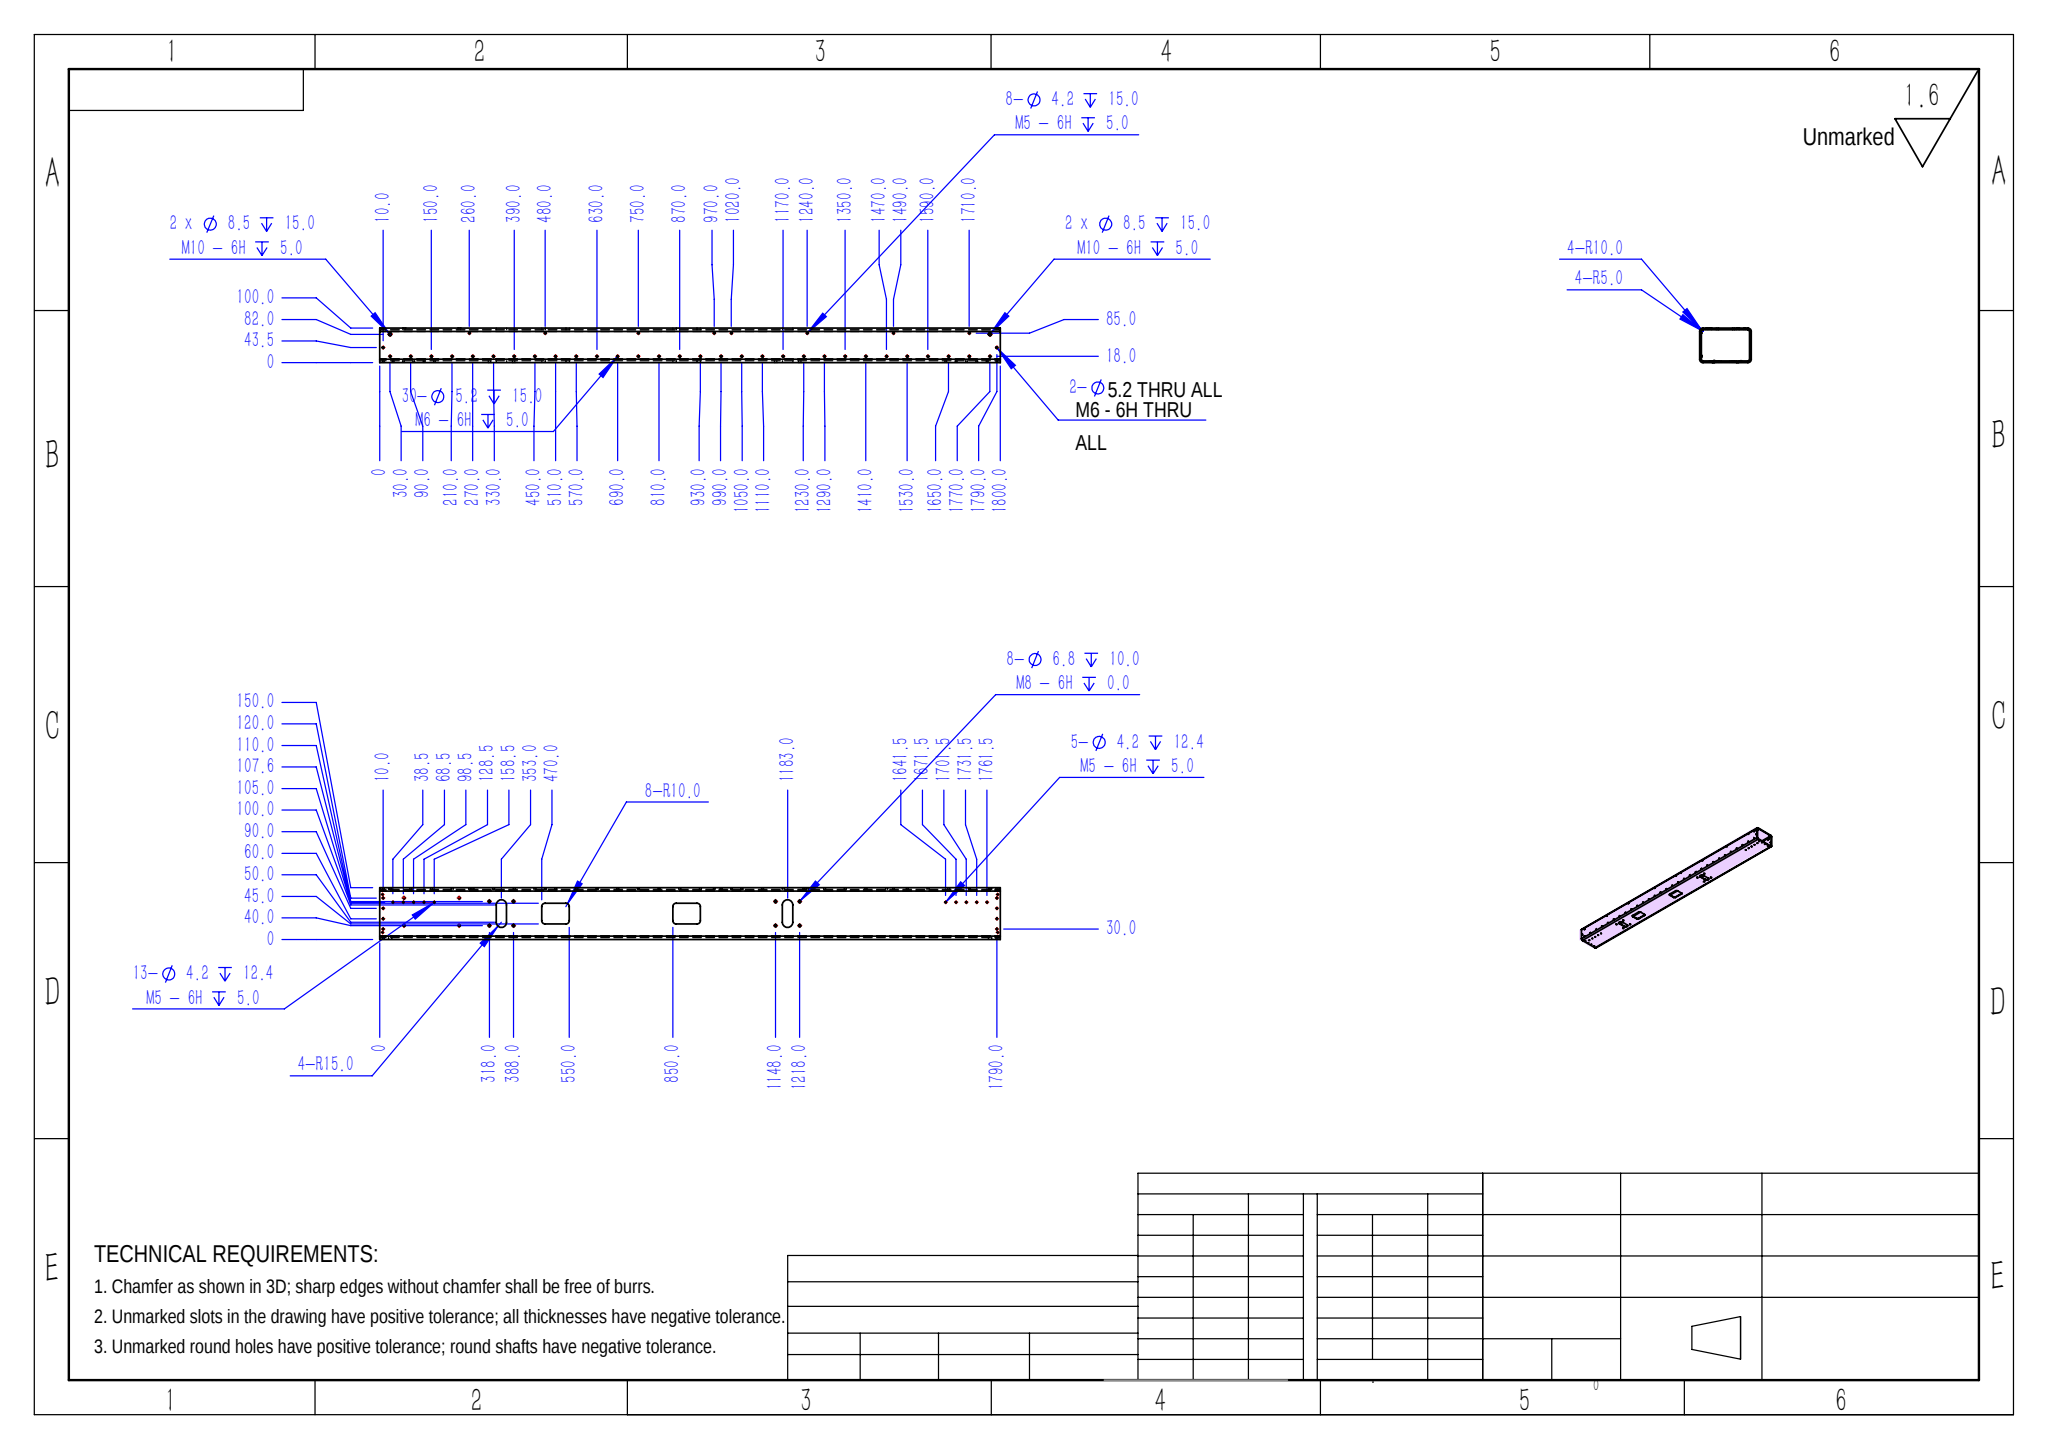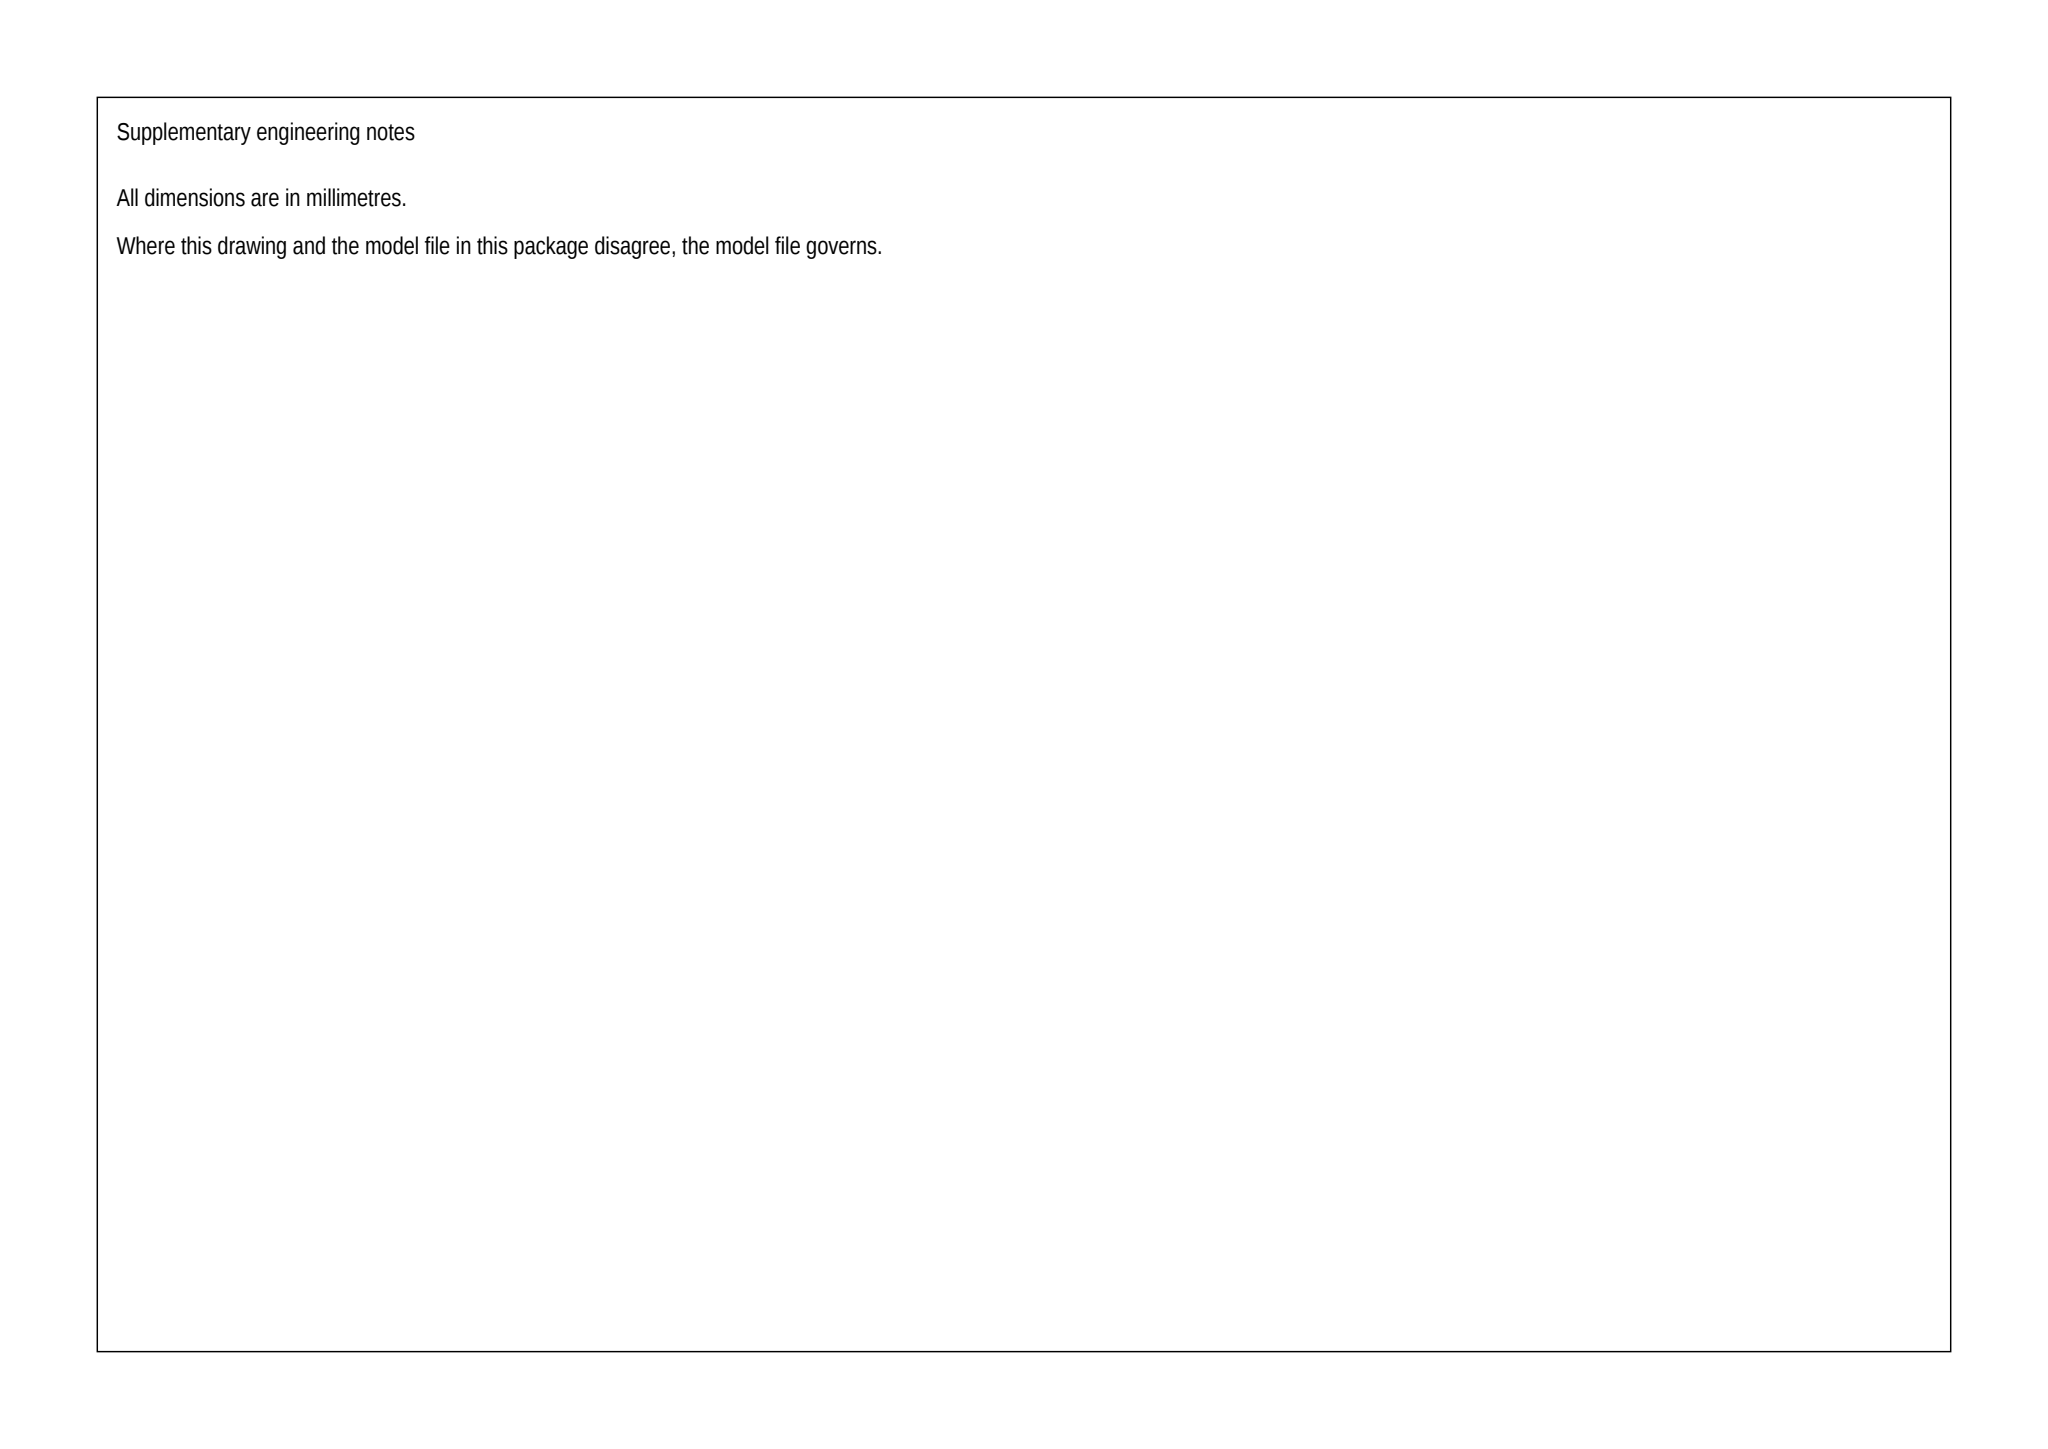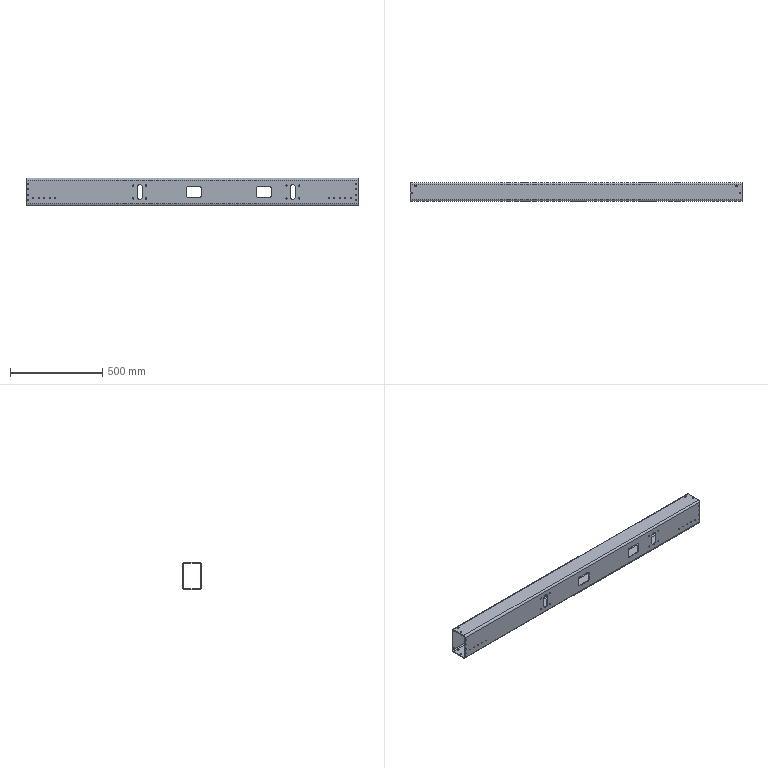Part | SolidWorks | mm | 1 solid | 226 faces | box 1800 x 100 x 150 mm | volume 4056692 mm3 | cylinder 192 | plane 34 | commonest cylinder face diameters 5.2 x68 4.2 x60 6.8 x24 20 x20 8.5 x8 30 x8 10 x4
Drawing notes:
SECT: 150 X 100 RECT TUBE, 1800 LG, WALL THK 5 ALL 4 SIDES | from the solid: bbox 1800x100x150; axis planes y=0/5/95/100 and z=0/5/145/150
4X Ø10 THRU 1800 LG, 10 FROM EA ADJACENT OUTER FACE | from the solid: cyl Ø10 axis x, len 1800 at (y,z)=(10,10),(10,140),(90,10),(90,140)
2X POCKET 80 LG X 60 HI, X 870-950 & 1250-1330, Z 45-105, THRU BOTH WALLS | from the solid: x planes 870/950 & 1250/1330 (cnt 2 ea); z planes 45/105 (cnt 4 ea); walls 5 THK
2X SIDE CUTOUT 30 LG X 60 HI, X 602-632 & 1432-1462, Z 45-105, THRU BOTH WALLS | from the solid: x planes 602/632 & 1432/1462 (cnt 2 ea); z planes 45/105; y planes 0,5,95,100
SIDE M5 ROWS X 38.5-158.5 & 1641.5-1761.5 AT Z=42.37 FROM BOT FACE | from the solid: Ø4.2 axis y at z=42.37, x=38.5..158.5 and 1641.5..1761.5
SIDE M5 AT X=10 & 1790: Z=30,60,90,120 FROM BOT FACE | from the solid: Ø4.2 axis y at x=10 & 1790, z=30,60,90,120
SIDE M5 AT X=8 & 1792: Z=20 & 130 FROM BOT FACE | from the solid: Ø4.2 axis y at x=8 & 1792, z=20 and 130
SIDE M8 (Ø6.8) AT X=582,652,1412,1482: Z=40 & 110 FROM BOT FACE | from the solid: Ø6.8 axis y at x=582,652,1412,1482, z=40 and 110
SIDE M8 (Ø6.8) AT X=1570 & 1730: Z=30 & 110 FROM BOT FACE | from the solid: Ø6.8 axis y at x=1570 & 1730, z=30 and 110
ALL SIDE-WALL HOLES 2X, BOTH WALLS (Y 0-5 & 95-100), DP 5 EA | from the solid: all axis-y cylinders count 2, length 5; walls y 0-5, 95-100
TOP 8X M5 AT Y=85: X=90,310,560,780,830,1050,1320,1540 | from the solid: Ø4.2 axis z at y=85, x=90,310,560,780,830,1050,1320,1540
ALL TOP-FACE HOLE PATTERNS REPEAT IN BTM WALL, DP 5 EA | from the solid: axis-z cylinders count 2 per position, length 5; walls z 0-5, 145-150
Ø5.2 DP 15 / M6-6H DP 5 AT X=10 & 1790: Y=43.5 & 56.5, TOP & BOT FACES | from the solid: cylinders [5.2,"z",[10.0,43.5,null],5.0,count 4] and [5.2,"z",[1790.0,43.5,null],5.0,count 4]; bbox Y=100 so mirrored row at Y=100-43.5=56.5; 4 per end = 2 Y-rows x 2 faces (z=0/150)
POCKETS 80x60 AT X=870 & 1250; CUTOUTS 30x60 AT X=602 & 1432 | from the solid: axis_planes x=870/950 & 1250/1330 (80 wide), x=602/632 & 1432/1462 (30 wide), z=45/105 count 4 (60 high)
build123d program:
from build123d import *

# Parameters (mm, degrees)
GB_6728_1986_RECTANGULAR_HOLLOW_SECTION_DEPTH = 1800
SKETCH2_W                                     = 80
SKETCH2_H                                     = 60
CUT_EXTRUDE1_DEPTH                            = 909.639
LPATTERN1_COUNT                               = 2
LPATTERN1_PITCH                               = 380
FILLET1_R                                     = 10
M6_TAPPED_HOLE1_D                             = 5.2
M5_TAPPED_HOLE1_AT_2_COUNT                    = 2
M5_TAPPED_HOLE1_AT_2_PITCH                    = 30
M5_TAPPED_HOLE1_AT_3_COUNT                    = 2
M5_TAPPED_HOLE1_AT_3_PITCH                    = 90
M5_TAPPED_HOLE1_AT_4_COUNT                    = 2
M5_TAPPED_HOLE1_AT_4_PITCH                    = 60
LPATTERN2_COUNT                               = 5
LPATTERN2_PITCH                               = 30
M10_TAPPED_HOLE1_D                            = 8.5
M10_TAPPED_HOLE1_DEPTH                        = 15
M10_TAPPED_HOLE1_TIP                          = 2.554
M8_TAPPED_HOLE3_D                             = 6.8
M8_TAPPED_HOLE3_DEPTH                         = 10
M8_TAPPED_HOLE3_TIP                           = 2.043
CUT_EXTRUDE2_DEPTH                            = 909.639
M5_TAPPED_HOLE5_D                             = 4.2
M5_TAPPED_HOLE5_DEPTH                         = 15
M5_TAPPED_HOLE5_TIP                           = 1.262
M6_TAPPED_HOLE2_D                             = 5.2
M6_TAPPED_HOLE2_DEPTH                         = 15
M6_TAPPED_HOLE2_TIP                           = 1.562
M8_TAPPED_HOLE5_D                             = 6.8
M8_TAPPED_HOLE5_DEPTH                         = 15
M8_TAPPED_HOLE5_TIP                           = 2.043
M5_TAPPED_HOLE6_AT_2_COUNT                    = 2
M5_TAPPED_HOLE6_AT_2_PITCH                    = 110


with BuildPart() as part:
    # Sketch11 → GB_6728-1986 Rectangular Hollow Section (new body)
    with BuildSketch(Plane.YZ.offset(-900)):
        with BuildLine():
            Line((-40, -75), (40, -75))
            ThreePointArc((40, -75), (47.071, -72.071), (50, -65))
            Line((50, -65), (50, 65))
            ThreePointArc((50, 65), (47.071, 72.071), (40, 75))
            Line((40, 75), (-40, 75))
            ThreePointArc((-40, 75), (-47.071, 72.071), (-50, 65))
            Line((-50, 65), (-50, -65))
            ThreePointArc((-50, -65), (-47.071, -72.071), (-40, -75))
        make_face()
        with BuildLine():
            Line((-40, -70), (40, -70))
            ThreePointArc((40, -70), (43.536, -68.536), (45, -65))
            Line((45, -65), (45, 65))
            ThreePointArc((45, 65), (43.536, 68.536), (40, 70))
            Line((40, 70), (-40, 70))
            ThreePointArc((-40, 70), (-43.536, 68.536), (-45, 65))
            Line((-45, 65), (-45, -65))
            ThreePointArc((-45, -65), (-43.536, -68.536), (-40, -70))
        make_face(mode=Mode.SUBTRACT)
    extrude(amount=GB_6728_1986_RECTANGULAR_HOLLOW_SECTION_DEPTH)

    # Sketch2 → Cut-Extrude1 (cut, through all)
    with BuildSketch(Plane.XZ.offset(50)):
        with Locations((390, 0)):
            Rectangle(SKETCH2_W, SKETCH2_H)
    cut_extrude1 = extrude(amount=-CUT_EXTRUDE1_DEPTH, mode=Mode.SUBTRACT)

    # LPattern1: Cut-Extrude1 ×2
    with Locations(*[(-i * LPATTERN1_PITCH, 0, 0) for i in range(1, LPATTERN1_COUNT)]):
        add(cut_extrude1, mode=Mode.SUBTRACT)

    # Fillet1
    fillet1_edges = [part.edges().sort_by_distance(p)[0] for p in [
        (430, 47.5, 30),
        (430, 47.5, -30),
        (350, 47.5, -30),
        (350, 47.5, 30),
        (430, -47.5, 30),
        (430, -47.5, -30),
        (350, -47.5, -30),
        (350, -47.5, 30),
        (50, 47.5, 30),
        (50, 47.5, -30),
        (-30, 47.5, -30),
        (-30, 47.5, 30),
        (50, -47.5, 30),
        (50, -47.5, -30),
        (-30, -47.5, -30),
        (-30, -47.5, 30),
    ]]
    fillet(fillet1_edges, radius=FILLET1_R)

    # M6 Tapped Hole1 (through all)
    with Locations(Plane.XY.offset(75)):
        with Locations((890, -6.5), (-890, -6.5)):
            Hole(M6_TAPPED_HOLE1_D / 2)

    # Sketch5 → M5 Tapped Hole1 (revolve, cut)
    with BuildSketch(Plane(origin=(890, -50, -45), x_dir=(0, 0, -1), z_dir=(1, 0, 0))):
        Polygon((0, 0), (0, 13.662), (2.1, 12.4), (2.1, 0), align=None)
    m5_tapped_hole1 = revolve(axis=Axis((890, -56.35, -45), (0, 1, 0)), mode=Mode.SUBTRACT)

    # M5 Tapped Hole1 at 2: M5 Tapped Hole1 ×2
    with Locations(*[(0, 0, i * M5_TAPPED_HOLE1_AT_2_PITCH) for i in range(1, M5_TAPPED_HOLE1_AT_2_COUNT)]):
        add(m5_tapped_hole1, mode=Mode.SUBTRACT)

    # M5 Tapped Hole1 at 3: M5 Tapped Hole1 ×2
    with Locations(*[(0, 0, i * M5_TAPPED_HOLE1_AT_3_PITCH) for i in range(1, M5_TAPPED_HOLE1_AT_3_COUNT)]):
        add(m5_tapped_hole1, mode=Mode.SUBTRACT)

    # M5 Tapped Hole1 at 4: M5 Tapped Hole1 ×2
    with Locations(*[(0, 0, i * M5_TAPPED_HOLE1_AT_4_PITCH) for i in range(1, M5_TAPPED_HOLE1_AT_4_COUNT)]):
        add(m5_tapped_hole1, mode=Mode.SUBTRACT)

    # Sketch8 → M5 Tapped Hole2 (revolve, cut)
    with BuildSketch(Plane(origin=(861.5, -50, -32.627), x_dir=(0, 0, -1), z_dir=(1, 0, 0))):
        Polygon((0, 0), (0, 13.662), (2.1, 12.4), (2.1, 0), align=None)
    m5_tapped_hole2 = revolve(axis=Axis((861.5, -56.35, -32.627), (0, 1, 0)), mode=Mode.SUBTRACT)

    # LPattern2: M5 Tapped Hole2 ×5
    with Locations(*[(-i * LPATTERN2_PITCH, 0, 0) for i in range(1, LPATTERN2_COUNT)]):
        add(m5_tapped_hole2, mode=Mode.SUBTRACT)

    # M10 Tapped Hole1
    with Locations(Plane(origin=(0, 0, 70), x_dir=(-1, 0, 0), z_dir=(0, 0, -1))):
        with Locations((-870, 32), (870, 32)):
            Hole(M10_TAPPED_HOLE1_D / 2, depth=M10_TAPPED_HOLE1_DEPTH)
            with Locations((0, 0, -(M10_TAPPED_HOLE1_DEPTH + M10_TAPPED_HOLE1_TIP / 2))):  # 118° drill point
                Cone(0, M10_TAPPED_HOLE1_D / 2, M10_TAPPED_HOLE1_TIP, mode=Mode.SUBTRACT)

    # Sketch11_2 → M10 Tapped Hole2 (revolve, cut)
    with BuildSketch(Plane(origin=(870, 32, -70), x_dir=(0, -1, 0), z_dir=(1, 0, 0))):
        Polygon((0, 0), (0, 17.554), (4.25, 15), (4.25, 0), align=None)
    m10_tapped_hole2 = revolve(axis=Axis((870, 32, -63.65), (0, 0, -1)), mode=Mode.SUBTRACT)

    # M8 Tapped Hole3
    with Locations(Plane(origin=(0, -50, 0), x_dir=(-1, 0, 0), z_dir=(0, -1, 0))):
        with Locations((-512, -35), (-582, -35), (-582, 35), (-512, 35), (318, -35), (248, -35), (248, 35), (318, 35)):
            Hole(M8_TAPPED_HOLE3_D / 2, depth=M8_TAPPED_HOLE3_DEPTH)
            with Locations((0, 0, -(M8_TAPPED_HOLE3_DEPTH + M8_TAPPED_HOLE3_TIP / 2))):  # 118° drill point
                Cone(0, M8_TAPPED_HOLE3_D / 2, M8_TAPPED_HOLE3_TIP, mode=Mode.SUBTRACT)

    # Sketch21 → Cut-Extrude2 (cut, through all)
    with BuildSketch(Plane.XZ.offset(50)):
        with BuildLine():
            Line((-298, 25), (-298, -25))
            ThreePointArc((-298, -25), (-283, -40), (-268, -25))
            Line((-268, -25), (-268, 25))
            ThreePointArc((-268, 25), (-283, 40), (-298, 25))
        make_face()
        with BuildLine():
            Line((532, 25), (532, -25))
            ThreePointArc((532, -25), (547, -40), (562, -25))
            Line((562, -25), (562, 25))
            ThreePointArc((562, 25), (547, 40), (532, 25))
        make_face()
    extrude(amount=-CUT_EXTRUDE2_DEPTH, mode=Mode.SUBTRACT)

    # Mirror1: M5 Tapped Hole2, M10 Tapped Hole2 across plane
    add(m5_tapped_hole2.mirror(Plane(origin=(0, 0, 0), x_dir=(0, 0, 1), z_dir=(1, 0, 0))), mode=Mode.SUBTRACT)
    add(m10_tapped_hole2.mirror(Plane(origin=(0, 0, 0), x_dir=(0, 0, 1), z_dir=(1, 0, 0))), mode=Mode.SUBTRACT)

    # Mirror1 copy 1 sketch → Mirror1 copy 1 (revolve, cut)
    with BuildSketch(Plane(origin=(-831.5, -50, -32.627), x_dir=(0, 0, -1), z_dir=(-1, 0, 0))):
        Polygon((0, 0), (0, -13.662), (2.1, -12.4), (2.1, 0), align=None)
    revolve(axis=Axis((-831.5, -56.35, -32.627), (0, -1, 0)), mode=Mode.SUBTRACT)

    # Mirror1 copy 2 sketch → Mirror1 copy 2 (revolve, cut)
    with BuildSketch(Plane(origin=(-801.5, -50, -32.627), x_dir=(0, 0, -1), z_dir=(-1, 0, 0))):
        Polygon((0, 0), (0, -13.662), (2.1, -12.4), (2.1, 0), align=None)
    revolve(axis=Axis((-801.5, -56.35, -32.627), (0, -1, 0)), mode=Mode.SUBTRACT)

    # Mirror1 copy 3 sketch → Mirror1 copy 3 (revolve, cut)
    with BuildSketch(Plane(origin=(-771.5, -50, -32.627), x_dir=(0, 0, -1), z_dir=(-1, 0, 0))):
        Polygon((0, 0), (0, -13.662), (2.1, -12.4), (2.1, 0), align=None)
    revolve(axis=Axis((-771.5, -56.35, -32.627), (0, -1, 0)), mode=Mode.SUBTRACT)

    # Mirror1 copy 4 sketch → Mirror1 copy 4 (revolve, cut)
    with BuildSketch(Plane(origin=(-741.5, -50, -32.627), x_dir=(0, 0, -1), z_dir=(-1, 0, 0))):
        Polygon((0, 0), (0, -13.662), (2.1, -12.4), (2.1, 0), align=None)
    revolve(axis=Axis((-741.5, -56.35, -32.627), (0, -1, 0)), mode=Mode.SUBTRACT)

    # M5 Tapped Hole5
    with Locations(Plane(origin=(0, 0, -75), x_dir=(-1, 0, 0), z_dir=(0, 0, -1))):
        with Locations((70, 35), (-150, 35), (-640, 35), (-420, 35), (810, 35), (590, 35), (120, 35), (340, 35)):
            Hole(M5_TAPPED_HOLE5_D / 2, depth=M5_TAPPED_HOLE5_DEPTH)
            with Locations((0, 0, -(M5_TAPPED_HOLE5_DEPTH + M5_TAPPED_HOLE5_TIP / 2))):  # 118° drill point
                Cone(0, M5_TAPPED_HOLE5_D / 2, M5_TAPPED_HOLE5_TIP, mode=Mode.SUBTRACT)

    # M6 Tapped Hole2
    with Locations(Plane(origin=(0, 0, -75), x_dir=(-1, 0, 0), z_dir=(0, 0, -1))):
        with Locations((870, -32), (-870, -32), (-810, -32), (-750, -32), (-690, -32), (-630, -32), (-570, -32), (-510, -32), (-450, -32), (-390, -32), (-330, -32), (-270, -32), (-210, -32), (-150, -32), (-90, -32), (-30, -32), (30, -32), (90, -32), (150, -32), (210, -32), (270, -32), (330, -32), (390, -32), (450, -32), (510, -32), (570, -32), (630, -32), (690, -32), (750, -32), (810, -32)):
            Hole(M6_TAPPED_HOLE2_D / 2, depth=M6_TAPPED_HOLE2_DEPTH)
            with Locations((0, 0, -(M6_TAPPED_HOLE2_DEPTH + M6_TAPPED_HOLE2_TIP / 2))):  # 118° drill point
                Cone(0, M6_TAPPED_HOLE2_D / 2, M6_TAPPED_HOLE2_TIP, mode=Mode.SUBTRACT)

    # M8 Tapped Hole5
    with Locations(Plane(origin=(0, 50, 0), x_dir=(1, 0, 0), z_dir=(0, 1, 0))):
        with Locations((670, 45), (670, -35), (830, 45), (830, -35)):
            Hole(M8_TAPPED_HOLE5_D / 2, depth=M8_TAPPED_HOLE5_DEPTH)
            with Locations((0, 0, -(M8_TAPPED_HOLE5_DEPTH + M8_TAPPED_HOLE5_TIP / 2))):  # 118° drill point
                Cone(0, M8_TAPPED_HOLE5_D / 2, M8_TAPPED_HOLE5_TIP, mode=Mode.SUBTRACT)

    # Mirror2: M5 Tapped Hole1 across plane
    add(m5_tapped_hole1.mirror(Plane(origin=(0, 0, 0), x_dir=(0, 0, 1), z_dir=(1, 0, 0))), mode=Mode.SUBTRACT)

    # Mirror2 copy 1 sketch → Mirror2 copy 1 (revolve, cut)
    with BuildSketch(Plane(origin=(-890, -50, -15), x_dir=(0, 0, -1), z_dir=(-1, 0, 0))):
        Polygon((0, 0), (0, -13.662), (2.1, -12.4), (2.1, 0), align=None)
    revolve(axis=Axis((-890, -56.35, -15), (0, -1, 0)), mode=Mode.SUBTRACT)

    # Mirror2 copy 2 sketch → Mirror2 copy 2 (revolve, cut)
    with BuildSketch(Plane(origin=(-890, -50, 45), x_dir=(0, 0, -1), z_dir=(-1, 0, 0))):
        Polygon((0, 0), (0, -13.662), (2.1, -12.4), (2.1, 0), align=None)
    revolve(axis=Axis((-890, -56.35, 45), (0, -1, 0)), mode=Mode.SUBTRACT)

    # Mirror2 copy 3 sketch → Mirror2 copy 3 (revolve, cut)
    with BuildSketch(Plane(origin=(-890, -50, 15), x_dir=(0, 0, -1), z_dir=(-1, 0, 0))):
        Polygon((0, 0), (0, -13.662), (2.1, -12.4), (2.1, 0), align=None)
    revolve(axis=Axis((-890, -56.35, 15), (0, -1, 0)), mode=Mode.SUBTRACT)

    # Sketch42 → M5 Tapped Hole6 (revolve, cut)
    with BuildSketch(Plane(origin=(892, 50, 55), x_dir=(0, 0, 1), z_dir=(1, 0, 0))):
        Polygon((0, 0), (0, 11.262), (2.1, 10), (2.1, 0), align=None)
    m5_tapped_hole6 = revolve(axis=Axis((892, 56.35, 55), (0, -1, 0)), mode=Mode.SUBTRACT)

    # M5 Tapped Hole6 at 2: M5 Tapped Hole6 ×2
    with Locations(*[(0, 0, -i * M5_TAPPED_HOLE6_AT_2_PITCH) for i in range(1, M5_TAPPED_HOLE6_AT_2_COUNT)]):
        add(m5_tapped_hole6, mode=Mode.SUBTRACT)

    # Mirror3: M5 Tapped Hole6 across plane
    add(m5_tapped_hole6.mirror(Plane(origin=(0, 0, 0), x_dir=(0, 0, 1), z_dir=(1, 0, 0))), mode=Mode.SUBTRACT)

    # Mirror3 copy 1 sketch → Mirror3 copy 1 (revolve, cut)
    with BuildSketch(Plane(origin=(-892, 50, -55), x_dir=(0, 0, 1), z_dir=(-1, 0, 0))):
        Polygon((0, 0), (0, -11.262), (2.1, -10), (2.1, 0), align=None)
    revolve(axis=Axis((-892, 56.35, -55), (0, 1, 0)), mode=Mode.SUBTRACT)


solid = part.part